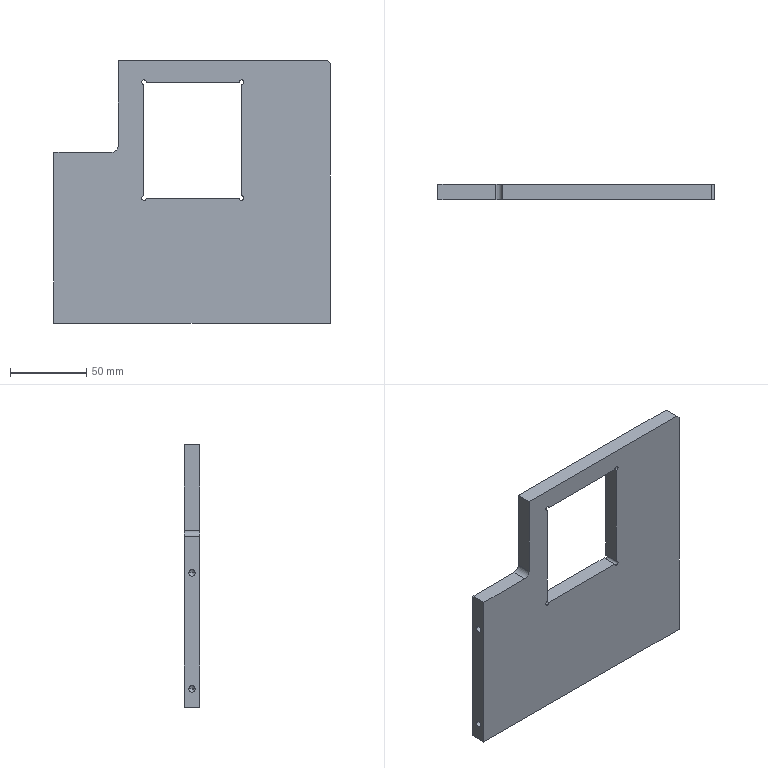Component | SolidWorks | AssemblyCylinderBracket54-1_GuideRailPlane-1 | 1 solid | 36 faces | box 181 x 10 x 172 mm | volume 236483 mm3 | cylinder 15 | plane 13 | cone 8 | commonest cylinder face diameters 4.2 x8 3 x6 8 x1
build123d program:
from build123d import *

# Parameters (mm, degrees)
SKETCH1_W                      = 172
SKETCH1_H                      = 181
BOSS_EXTRUDE1_DEPTH            = 10
CHAMFER1_SIZE                  = 2
M5X0_8_TAPPED_HOLE1_AT_2_COUNT = 2
M5X0_8_TAPPED_HOLE1_AT_2_PITCH = 76
SKETCH13_W                     = 60
SKETCH13_H                     = 42
CUT_EXTRUDE1_DEPTH             = 10
FILLET1_R                      = 4
SKETCH14_W                     = 76
SKETCH14_H                     = 64
CUT_EXTRUDE2_DEPTH             = 126.245
SKETCH15_R                     = 1.5
CUT_EXTRUDE3_DEPTH             = 10


with BuildPart() as part:
    # Sketch1 → Boss-Extrude1 (new body)
    with BuildSketch(Plane.XY):
        Rectangle(SKETCH1_W, SKETCH1_H)
    extrude(amount=BOSS_EXTRUDE1_DEPTH)

    # Chamfer1
    chamfer1_edges = [part.edges().sort_by_distance(p)[0] for p in [
        (86, -90.5, 5),
        (86, 90.5, 5),
    ]]
    chamfer(chamfer1_edges, length=CHAMFER1_SIZE)

    # Sketch6 → M5x0.8 Tapped Hole1 (revolve, cut)
    with BuildSketch(Plane(origin=(-74, -90.5, 5), x_dir=(0, 0, -1), z_dir=(1, 0, 0))):
        Polygon((0, 0), (0, 15.262), (2.1, 14), (2.1, 0), align=None)
    m5x0_8_tapped_hole1 = revolve(axis=Axis((-74, -96.85, 5), (0, 1, 0)), mode=Mode.SUBTRACT)

    # M5x0.8 Tapped Hole1 at 2: M5x0.8 Tapped Hole1 ×2
    with Locations(*[(i * M5X0_8_TAPPED_HOLE1_AT_2_PITCH, 0, 0) for i in range(1, M5X0_8_TAPPED_HOLE1_AT_2_COUNT)]):
        add(m5x0_8_tapped_hole1, mode=Mode.SUBTRACT)

    # Mirror1: M5x0.8 Tapped Hole1 across plane
    add(m5x0_8_tapped_hole1.mirror(Plane.ZX), mode=Mode.SUBTRACT)

    # Mirror1 copy 1 sketch → Mirror1 copy 1 (revolve, cut)
    with BuildSketch(Plane(origin=(2, 90.5, 5), x_dir=(0, 0, -1), z_dir=(1, 0, 0))):
        Polygon((0, 0), (0, -15.262), (2.1, -14), (2.1, 0), align=None)
    revolve(axis=Axis((2, 96.85, 5), (0, 1, 0)), mode=Mode.SUBTRACT)

    # Sketch13 → Cut-Extrude1 (cut)
    with BuildSketch(Plane.XY.offset(10)):
        with Locations((56, -69.5)):
            Rectangle(SKETCH13_W, SKETCH13_H)
    extrude(amount=-CUT_EXTRUDE1_DEPTH, mode=Mode.SUBTRACT)

    # Fillet1
    fillet1_edges = [part.edges().sort_by_distance(p)[0] for p in [
        (26, -48.5, 5),
    ]]
    fillet(fillet1_edges, radius=FILLET1_R)

    # Sketch14 → Cut-Extrude2 (cut, through all)
    with BuildSketch(Plane.XY.offset(10)):
        with Locations((34, 0.5)):
            Rectangle(SKETCH14_W, SKETCH14_H)
    extrude(amount=-CUT_EXTRUDE2_DEPTH, mode=Mode.SUBTRACT)

    # Sketch15 → Cut-Extrude3 (cut)
    with BuildSketch(Plane.XY.offset(10)):
        with Locations((-4, 32.5)):
            Circle(SKETCH15_R)
        with Locations((72, 32.5)):
            Circle(SKETCH15_R)
        with Locations((72, -31.5)):
            Circle(SKETCH15_R)
        with Locations((-4, -31.5)):
            Circle(SKETCH15_R)
    extrude(amount=-CUT_EXTRUDE3_DEPTH, mode=Mode.SUBTRACT)


solid = part.part

# Placed as in the assembly
solid = solid.moved(Location((54.585, -11.305, 87.359), (-90, 0, -90)))
STEP:
#1=COLOUR_RGB('',0.7922,0.8196,0.9333);
#2=FILL_AREA_STYLE_COLOUR('',#1);
#3=FILL_AREA_STYLE('',(#2));
#4=SURFACE_STYLE_FILL_AREA(#3);
#5=SURFACE_SIDE_STYLE('',(#4));
#6=SURFACE_STYLE_USAGE(.BOTH.,#5);
#7=PRESENTATION_STYLE_ASSIGNMENT((#6));
#8=CARTESIAN_POINT('',(0.9089,-0.4451,6.333));
#9=VERTEX_POINT('',#8);
#10=CARTESIAN_POINT('',(0.9679,-0.4451,6.274));
#11=VERTEX_POINT('',#10);
#12=CARTESIAN_POINT('',(0.9089,-0.4451,6.274));
#13=DIRECTION('',(-0.,1.,-0.));
#14=DIRECTION('',(0.,0.,1.));
#15=AXIS2_PLACEMENT_3D('',#12,#13,#14);
#16=CIRCLE('',#15,0.05906);
#17=EDGE_CURVE('',#9,#11,#16,.T.);
#18=ORIENTED_EDGE('',*,*,#17,.F.);
#19=CARTESIAN_POINT('',(0.9089,-0.05139,6.333));
#20=VERTEX_POINT('',#19);
#21=CARTESIAN_POINT('',(0.9089,-0.4451,6.333));
#22=DIRECTION('',(-0.,1.,-0.));
#23=VECTOR('',#22,39.37);
#24=LINE('',#21,#23);
#25=EDGE_CURVE('',#9,#20,#24,.T.);
#26=ORIENTED_EDGE('',*,*,#25,.T.);
#27=CARTESIAN_POINT('',(0.9679,-0.05139,6.274));
#28=VERTEX_POINT('',#27);
#29=CARTESIAN_POINT('',(0.9089,-0.05139,6.274));
#30=DIRECTION('',(-0.,1.,-0.));
#31=DIRECTION('',(0.,0.,1.));
#32=AXIS2_PLACEMENT_3D('',#29,#30,#31);
#33=CIRCLE('',#32,0.05906);
#34=EDGE_CURVE('',#20,#28,#33,.T.);
#35=ORIENTED_EDGE('',*,*,#34,.T.);
#36=CARTESIAN_POINT('',(0.9679,-0.4451,6.274));
#37=DIRECTION('',(-0.,1.,-0.));
#38=VECTOR('',#37,39.37);
#39=LINE('',#36,#38);
#40=EDGE_CURVE('',#11,#28,#39,.T.);
#41=ORIENTED_EDGE('',*,*,#40,.F.);
#42=EDGE_LOOP('',(#18,#26,#35,#41));
#43=FACE_OUTER_BOUND('',#42,.T.);
#44=CARTESIAN_POINT('',(0.9089,-0.4451,6.274));
#45=DIRECTION('',(-0.,1.,-0.));
#46=DIRECTION('',(0.,0.,1.));
#47=AXIS2_PLACEMENT_3D('',#44,#45,#46);
#48=CYLINDRICAL_SURFACE('',#47,0.05906);
#49=ADVANCED_FACE('',(#43),#48,.F.);
#50=CARTESIAN_POINT('',(3.429,-0.4451,6.333));
#51=VERTEX_POINT('',#50);
#52=CARTESIAN_POINT('',(3.429,-0.4451,6.215));
#53=VERTEX_POINT('',#52);
#54=CARTESIAN_POINT('',(3.429,-0.4451,6.274));
#55=DIRECTION('',(-0.,1.,-0.));
#56=DIRECTION('',(0.,0.,1.));
#57=AXIS2_PLACEMENT_3D('',#54,#55,#56);
#58=CIRCLE('',#57,0.05906);
#59=EDGE_CURVE('',#51,#53,#58,.T.);
#60=ORIENTED_EDGE('',*,*,#59,.F.);
#61=CARTESIAN_POINT('',(3.429,-0.05139,6.333));
#62=VERTEX_POINT('',#61);
#63=CARTESIAN_POINT('',(3.429,-0.4451,6.333));
#64=DIRECTION('',(-0.,1.,-0.));
#65=VECTOR('',#64,39.37);
#66=LINE('',#63,#65);
#67=EDGE_CURVE('',#51,#62,#66,.T.);
#68=ORIENTED_EDGE('',*,*,#67,.T.);
#69=CARTESIAN_POINT('',(3.429,-0.05139,6.215));
#70=VERTEX_POINT('',#69);
#71=CARTESIAN_POINT('',(3.429,-0.05139,6.274));
#72=DIRECTION('',(-0.,1.,-0.));
#73=DIRECTION('',(0.,0.,1.));
#74=AXIS2_PLACEMENT_3D('',#71,#72,#73);
#75=CIRCLE('',#74,0.05906);
#76=EDGE_CURVE('',#62,#70,#75,.T.);
#77=ORIENTED_EDGE('',*,*,#76,.T.);
#78=CARTESIAN_POINT('',(3.429,-0.4451,6.215));
#79=DIRECTION('',(-0.,1.,-0.));
#80=VECTOR('',#79,39.37);
#81=LINE('',#78,#80);
#82=EDGE_CURVE('',#53,#70,#81,.T.);
#83=ORIENTED_EDGE('',*,*,#82,.F.);
#84=EDGE_LOOP('',(#60,#68,#77,#83));
#85=FACE_OUTER_BOUND('',#84,.T.);
#86=CARTESIAN_POINT('',(3.429,-0.4451,6.274));
#87=DIRECTION('',(-0.,1.,-0.));
#88=DIRECTION('',(0.,0.,1.));
#89=AXIS2_PLACEMENT_3D('',#86,#87,#88);
#90=CYLINDRICAL_SURFACE('',#89,0.05906);
#91=ADVANCED_FACE('',(#85),#90,.F.);
#92=CARTESIAN_POINT('',(5.161,-0.3309,0.5259));
#93=VERTEX_POINT('',#92);
#94=CARTESIAN_POINT('',(5.161,-0.1656,0.5259));
#95=VERTEX_POINT('',#94);
#96=CARTESIAN_POINT('',(5.161,-0.2482,0.5259));
#97=DIRECTION('',(1.,-0.,0.));
#98=DIRECTION('',(0.,1.,0.));
#99=AXIS2_PLACEMENT_3D('',#96,#97,#98);
#100=CIRCLE('',#99,0.08268);
#101=EDGE_CURVE('',#93,#95,#100,.T.);
#102=ORIENTED_EDGE('',*,*,#101,.F.);
#103=CARTESIAN_POINT('',(5.712,-0.3309,0.5259));
#104=VERTEX_POINT('',#103);
#105=CARTESIAN_POINT('',(5.712,-0.3309,0.5259));
#106=DIRECTION('',(1.,-0.,0.));
#107=VECTOR('',#106,39.37);
#108=LINE('',#105,#107);
#109=EDGE_CURVE('',#93,#104,#108,.T.);
#110=ORIENTED_EDGE('',*,*,#109,.T.);
#111=CARTESIAN_POINT('',(5.712,-0.1656,0.5259));
#112=VERTEX_POINT('',#111);
#113=CARTESIAN_POINT('',(5.712,-0.2482,0.5259));
#114=DIRECTION('',(1.,-0.,0.));
#115=DIRECTION('',(0.,1.,0.));
#116=AXIS2_PLACEMENT_3D('',#113,#114,#115);
#117=CIRCLE('',#116,0.08268);
#118=EDGE_CURVE('',#104,#112,#117,.T.);
#119=ORIENTED_EDGE('',*,*,#118,.T.);
#120=CARTESIAN_POINT('',(5.712,-0.1656,0.5259));
#121=DIRECTION('',(1.,-0.,0.));
#122=VECTOR('',#121,39.37);
#123=LINE('',#120,#122);
#124=EDGE_CURVE('',#95,#112,#123,.T.);
#125=ORIENTED_EDGE('',*,*,#124,.F.);
#126=EDGE_LOOP('',(#102,#110,#119,#125));
#127=FACE_OUTER_BOUND('',#126,.T.);
#128=CARTESIAN_POINT('',(5.712,-0.2482,0.5259));
#129=DIRECTION('',(1.,-0.,0.));
#130=DIRECTION('',(0.,1.,0.));
#131=AXIS2_PLACEMENT_3D('',#128,#129,#130);
#132=CYLINDRICAL_SURFACE('',#131,0.08268);
#133=ADVANCED_FACE('',(#127),#132,.F.);
#134=CARTESIAN_POINT('',(5.111,-0.2482,0.5259));
#135=VERTEX_POINT('',#134);
#136=CARTESIAN_POINT('',(5.161,-0.1656,0.5259));
#137=DIRECTION('',(0.515,0.8572,0.));
#138=VECTOR('',#137,39.37);
#139=LINE('',#136,#138);
#140=EDGE_CURVE('',#135,#95,#139,.T.);
#141=ORIENTED_EDGE('',*,*,#140,.F.);
#142=CARTESIAN_POINT('',(5.161,-0.3309,0.5259));
#143=DIRECTION('',(0.515,-0.8572,0.));
#144=VECTOR('',#143,39.37);
#145=LINE('',#142,#144);
#146=EDGE_CURVE('',#135,#93,#145,.T.);
#147=ORIENTED_EDGE('',*,*,#146,.T.);
#148=ORIENTED_EDGE('',*,*,#101,.T.);
#149=EDGE_LOOP('',(#141,#147,#148));
#150=FACE_OUTER_BOUND('',#149,.T.);
#151=CARTESIAN_POINT('',(5.161,-0.2482,0.5259));
#152=DIRECTION('',(1.,-0.,0.));
#153=DIRECTION('',(0.,1.,0.));
#154=AXIS2_PLACEMENT_3D('',#151,#152,#153);
#155=CONICAL_SURFACE('',#154,0.08268,1.03);
#156=ADVANCED_FACE('',(#150),#155,.F.);
#157=CARTESIAN_POINT('',(5.161,-0.3309,3.518));
#158=VERTEX_POINT('',#157);
#159=CARTESIAN_POINT('',(5.161,-0.1656,3.518));
#160=VERTEX_POINT('',#159);
#161=CARTESIAN_POINT('',(5.161,-0.2482,3.518));
#162=DIRECTION('',(1.,-0.,0.));
#163=DIRECTION('',(0.,1.,0.));
#164=AXIS2_PLACEMENT_3D('',#161,#162,#163);
#165=CIRCLE('',#164,0.08268);
#166=EDGE_CURVE('',#158,#160,#165,.T.);
#167=ORIENTED_EDGE('',*,*,#166,.F.);
#168=CARTESIAN_POINT('',(5.712,-0.3309,3.518));
#169=VERTEX_POINT('',#168);
#170=CARTESIAN_POINT('',(5.712,-0.3309,3.518));
#171=DIRECTION('',(1.,-0.,0.));
#172=VECTOR('',#171,39.37);
#173=LINE('',#170,#172);
#174=EDGE_CURVE('',#158,#169,#173,.T.);
#175=ORIENTED_EDGE('',*,*,#174,.T.);
#176=CARTESIAN_POINT('',(5.712,-0.1656,3.518));
#177=VERTEX_POINT('',#176);
#178=CARTESIAN_POINT('',(5.712,-0.2482,3.518));
#179=DIRECTION('',(1.,-0.,0.));
#180=DIRECTION('',(0.,1.,0.));
#181=AXIS2_PLACEMENT_3D('',#178,#179,#180);
#182=CIRCLE('',#181,0.08268);
#183=EDGE_CURVE('',#169,#177,#182,.T.);
#184=ORIENTED_EDGE('',*,*,#183,.T.);
#185=CARTESIAN_POINT('',(5.712,-0.1656,3.518));
#186=DIRECTION('',(1.,-0.,0.));
#187=VECTOR('',#186,39.37);
#188=LINE('',#185,#187);
#189=EDGE_CURVE('',#160,#177,#188,.T.);
#190=ORIENTED_EDGE('',*,*,#189,.F.);
#191=EDGE_LOOP('',(#167,#175,#184,#190));
#192=FACE_OUTER_BOUND('',#191,.T.);
#193=CARTESIAN_POINT('',(5.712,-0.2482,3.518));
#194=DIRECTION('',(1.,-0.,0.));
#195=DIRECTION('',(0.,1.,0.));
#196=AXIS2_PLACEMENT_3D('',#193,#194,#195);
#197=CYLINDRICAL_SURFACE('',#196,0.08268);
#198=ADVANCED_FACE('',(#192),#197,.F.);
#199=CARTESIAN_POINT('',(5.111,-0.2482,3.518));
#200=VERTEX_POINT('',#199);
#201=CARTESIAN_POINT('',(5.161,-0.1656,3.518));
#202=DIRECTION('',(0.515,0.8572,0.));
#203=VECTOR('',#202,39.37);
#204=LINE('',#201,#203);
#205=EDGE_CURVE('',#200,#160,#204,.T.);
#206=ORIENTED_EDGE('',*,*,#205,.F.);
#207=CARTESIAN_POINT('',(5.161,-0.3309,3.518));
#208=DIRECTION('',(0.515,-0.8572,0.));
#209=VECTOR('',#208,39.37);
#210=LINE('',#207,#209);
#211=EDGE_CURVE('',#200,#158,#210,.T.);
#212=ORIENTED_EDGE('',*,*,#211,.T.);
#213=ORIENTED_EDGE('',*,*,#166,.T.);
#214=EDGE_LOOP('',(#206,#212,#213));
#215=FACE_OUTER_BOUND('',#214,.T.);
#216=CARTESIAN_POINT('',(5.161,-0.2482,3.518));
#217=DIRECTION('',(1.,-0.,0.));
#218=DIRECTION('',(0.,1.,0.));
#219=AXIS2_PLACEMENT_3D('',#216,#217,#218);
#220=CONICAL_SURFACE('',#219,0.08268,1.03);
#221=ADVANCED_FACE('',(#215),#220,.F.);
#222=CARTESIAN_POINT('',(-0.8628,-0.1656,0.5259));
#223=VERTEX_POINT('',#222);
#224=CARTESIAN_POINT('',(-0.8628,-0.3309,0.5259));
#225=VERTEX_POINT('',#224);
#226=CARTESIAN_POINT('',(-0.8628,-0.2482,0.5259));
#227=DIRECTION('',(-1.,0.,-0.));
#228=DIRECTION('',(0.,-1.,0.));
#229=AXIS2_PLACEMENT_3D('',#226,#227,#228);
#230=CIRCLE('',#229,0.08268);
#231=EDGE_CURVE('',#223,#225,#230,.T.);
#232=ORIENTED_EDGE('',*,*,#231,.F.);
#233=CARTESIAN_POINT('',(-1.414,-0.1656,0.5259));
#234=VERTEX_POINT('',#233);
#235=CARTESIAN_POINT('',(-1.414,-0.1656,0.5259));
#236=DIRECTION('',(-1.,0.,-0.));
#237=VECTOR('',#236,39.37);
#238=LINE('',#235,#237);
#239=EDGE_CURVE('',#223,#234,#238,.T.);
#240=ORIENTED_EDGE('',*,*,#239,.T.);
#241=CARTESIAN_POINT('',(-1.414,-0.3309,0.5259));
#242=VERTEX_POINT('',#241);
#243=CARTESIAN_POINT('',(-1.414,-0.2482,0.5259));
#244=DIRECTION('',(-1.,0.,-0.));
#245=DIRECTION('',(0.,-1.,0.));
#246=AXIS2_PLACEMENT_3D('',#243,#244,#245);
#247=CIRCLE('',#246,0.08268);
#248=EDGE_CURVE('',#234,#242,#247,.T.);
#249=ORIENTED_EDGE('',*,*,#248,.T.);
#250=CARTESIAN_POINT('',(-1.414,-0.3309,0.5259));
#251=DIRECTION('',(-1.,0.,-0.));
#252=VECTOR('',#251,39.37);
#253=LINE('',#250,#252);
#254=EDGE_CURVE('',#225,#242,#253,.T.);
#255=ORIENTED_EDGE('',*,*,#254,.F.);
#256=EDGE_LOOP('',(#232,#240,#249,#255));
#257=FACE_OUTER_BOUND('',#256,.T.);
#258=CARTESIAN_POINT('',(-1.414,-0.2482,0.5259));
#259=DIRECTION('',(-1.,0.,-0.));
#260=DIRECTION('',(0.,-1.,0.));
#261=AXIS2_PLACEMENT_3D('',#258,#259,#260);
#262=CYLINDRICAL_SURFACE('',#261,0.08268);
#263=ADVANCED_FACE('',(#257),#262,.F.);
#264=CARTESIAN_POINT('',(-0.8131,-0.2482,0.5259));
#265=VERTEX_POINT('',#264);
#266=CARTESIAN_POINT('',(-0.8628,-0.3309,0.5259));
#267=DIRECTION('',(-0.515,-0.8572,-0.));
#268=VECTOR('',#267,39.37);
#269=LINE('',#266,#268);
#270=EDGE_CURVE('',#265,#225,#269,.T.);
#271=ORIENTED_EDGE('',*,*,#270,.F.);
#272=CARTESIAN_POINT('',(-0.8628,-0.1656,0.5259));
#273=DIRECTION('',(-0.515,0.8572,0.));
#274=VECTOR('',#273,39.37);
#275=LINE('',#272,#274);
#276=EDGE_CURVE('',#265,#223,#275,.T.);
#277=ORIENTED_EDGE('',*,*,#276,.T.);
#278=ORIENTED_EDGE('',*,*,#231,.T.);
#279=EDGE_LOOP('',(#271,#277,#278));
#280=FACE_OUTER_BOUND('',#279,.T.);
#281=CARTESIAN_POINT('',(-0.8628,-0.2482,0.5259));
#282=DIRECTION('',(-1.,0.,-0.));
#283=DIRECTION('',(0.,-1.,0.));
#284=AXIS2_PLACEMENT_3D('',#281,#282,#283);
#285=CONICAL_SURFACE('',#284,0.08268,1.03);
#286=ADVANCED_FACE('',(#280),#285,.F.);
#287=CARTESIAN_POINT('',(-0.8628,-0.1656,3.518));
#288=VERTEX_POINT('',#287);
#289=CARTESIAN_POINT('',(-0.8628,-0.3309,3.518));
#290=VERTEX_POINT('',#289);
#291=CARTESIAN_POINT('',(-0.8628,-0.2482,3.518));
#292=DIRECTION('',(-1.,0.,-0.));
#293=DIRECTION('',(0.,-1.,0.));
#294=AXIS2_PLACEMENT_3D('',#291,#292,#293);
#295=CIRCLE('',#294,0.08268);
#296=EDGE_CURVE('',#288,#290,#295,.T.);
#297=ORIENTED_EDGE('',*,*,#296,.F.);
#298=CARTESIAN_POINT('',(-1.414,-0.1656,3.518));
#299=VERTEX_POINT('',#298);
#300=CARTESIAN_POINT('',(-1.414,-0.1656,3.518));
#301=DIRECTION('',(-1.,0.,-0.));
#302=VECTOR('',#301,39.37);
#303=LINE('',#300,#302);
#304=EDGE_CURVE('',#288,#299,#303,.T.);
#305=ORIENTED_EDGE('',*,*,#304,.T.);
#306=CARTESIAN_POINT('',(-1.414,-0.3309,3.518));
#307=VERTEX_POINT('',#306);
#308=CARTESIAN_POINT('',(-1.414,-0.2482,3.518));
#309=DIRECTION('',(-1.,0.,-0.));
#310=DIRECTION('',(0.,-1.,0.));
#311=AXIS2_PLACEMENT_3D('',#308,#309,#310);
#312=CIRCLE('',#311,0.08268);
#313=EDGE_CURVE('',#299,#307,#312,.T.);
#314=ORIENTED_EDGE('',*,*,#313,.T.);
#315=CARTESIAN_POINT('',(-1.414,-0.3309,3.518));
#316=DIRECTION('',(-1.,0.,-0.));
#317=VECTOR('',#316,39.37);
#318=LINE('',#315,#317);
#319=EDGE_CURVE('',#290,#307,#318,.T.);
#320=ORIENTED_EDGE('',*,*,#319,.F.);
#321=EDGE_LOOP('',(#297,#305,#314,#320));
#322=FACE_OUTER_BOUND('',#321,.T.);
#323=CARTESIAN_POINT('',(-1.414,-0.2482,3.518));
#324=DIRECTION('',(-1.,0.,-0.));
#325=DIRECTION('',(0.,-1.,0.));
#326=AXIS2_PLACEMENT_3D('',#323,#324,#325);
#327=CYLINDRICAL_SURFACE('',#326,0.08268);
#328=ADVANCED_FACE('',(#322),#327,.F.);
#329=CARTESIAN_POINT('',(-0.8131,-0.2482,3.518));
#330=VERTEX_POINT('',#329);
#331=CARTESIAN_POINT('',(-0.8628,-0.3309,3.518));
#332=DIRECTION('',(-0.515,-0.8572,-0.));
#333=VECTOR('',#332,39.37);
#334=LINE('',#331,#333);
#335=EDGE_CURVE('',#330,#290,#334,.T.);
#336=ORIENTED_EDGE('',*,*,#335,.F.);
#337=CARTESIAN_POINT('',(-0.8628,-0.1656,3.518));
#338=DIRECTION('',(-0.515,0.8572,0.));
#339=VECTOR('',#338,39.37);
#340=LINE('',#337,#339);
#341=EDGE_CURVE('',#330,#288,#340,.T.);
#342=ORIENTED_EDGE('',*,*,#341,.T.);
#343=ORIENTED_EDGE('',*,*,#296,.T.);
#344=EDGE_LOOP('',(#336,#342,#343));
#345=FACE_OUTER_BOUND('',#344,.T.);
#346=CARTESIAN_POINT('',(-0.8628,-0.2482,3.518));
#347=DIRECTION('',(-1.,0.,-0.));
#348=DIRECTION('',(0.,-1.,0.));
#349=AXIS2_PLACEMENT_3D('',#346,#347,#348);
#350=CONICAL_SURFACE('',#349,0.08268,1.03);
#351=ADVANCED_FACE('',(#345),#350,.F.);
#352=CARTESIAN_POINT('',(0.2396,-0.05139,6.825));
#353=VERTEX_POINT('',#352);
#354=CARTESIAN_POINT('',(5.633,-0.05139,6.825));
#355=VERTEX_POINT('',#354);
#356=CARTESIAN_POINT('',(5.712,-0.05139,6.825));
#357=DIRECTION('',(1.,-0.,-0.));
#358=VECTOR('',#357,39.37);
#359=LINE('',#356,#358);
#360=EDGE_CURVE('',#353,#355,#359,.T.);
#361=ORIENTED_EDGE('',*,*,#360,.F.);
#362=CARTESIAN_POINT('',(0.2396,-0.4451,6.825));
#363=VERTEX_POINT('',#362);
#364=CARTESIAN_POINT('',(0.2396,-0.4451,6.825));
#365=DIRECTION('',(-0.,1.,-0.));
#366=VECTOR('',#365,39.37);
#367=LINE('',#364,#366);
#368=EDGE_CURVE('',#363,#353,#367,.T.);
#369=ORIENTED_EDGE('',*,*,#368,.F.);
#370=CARTESIAN_POINT('',(5.633,-0.4451,6.825));
#371=VERTEX_POINT('',#370);
#372=CARTESIAN_POINT('',(5.712,-0.4451,6.825));
#373=DIRECTION('',(1.,-0.,-0.));
#374=VECTOR('',#373,39.37);
#375=LINE('',#372,#374);
#376=EDGE_CURVE('',#363,#371,#375,.T.);
#377=ORIENTED_EDGE('',*,*,#376,.T.);
#378=CARTESIAN_POINT('',(5.633,-0.05139,6.825));
#379=DIRECTION('',(-0.,1.,-0.));
#380=VECTOR('',#379,39.37);
#381=LINE('',#378,#380);
#382=EDGE_CURVE('',#371,#355,#381,.T.);
#383=ORIENTED_EDGE('',*,*,#382,.T.);
#384=EDGE_LOOP('',(#361,#369,#377,#383));
#385=FACE_OUTER_BOUND('',#384,.T.);
#386=CARTESIAN_POINT('',(5.712,-0.05139,6.825));
#387=DIRECTION('',(-0.,0.,-1.));
#388=DIRECTION('',(-1.,0.,0.));
#389=AXIS2_PLACEMENT_3D('',#386,#387,#388);
#390=PLANE('',#389);
#391=ADVANCED_FACE('',(#385),#390,.F.);
#392=CARTESIAN_POINT('',(5.712,-0.2482,0.5259));
#393=DIRECTION('',(1.,-0.,0.));
#394=DIRECTION('',(0.,1.,0.));
#395=AXIS2_PLACEMENT_3D('',#392,#393,#394);
#396=CIRCLE('',#395,0.08268);
#397=EDGE_CURVE('',#112,#104,#396,.T.);
#398=ORIENTED_EDGE('',*,*,#397,.F.);
#399=ORIENTED_EDGE('',*,*,#118,.F.);
#400=EDGE_LOOP('',(#398,#399));
#401=FACE_BOUND('',#400,.T.);
#402=CARTESIAN_POINT('',(5.712,-0.2482,3.518));
#403=DIRECTION('',(1.,-0.,0.));
#404=DIRECTION('',(0.,1.,0.));
#405=AXIS2_PLACEMENT_3D('',#402,#403,#404);
#406=CIRCLE('',#405,0.08268);
#407=EDGE_CURVE('',#177,#169,#406,.T.);
#408=ORIENTED_EDGE('',*,*,#407,.F.);
#409=ORIENTED_EDGE('',*,*,#183,.F.);
#410=EDGE_LOOP('',(#408,#409));
#411=FACE_BOUND('',#410,.T.);
#412=CARTESIAN_POINT('',(5.712,-0.05139,6.746));
#413=VERTEX_POINT('',#412);
#414=CARTESIAN_POINT('',(5.712,-0.05139,0.0535));
#415=VERTEX_POINT('',#414);
#416=CARTESIAN_POINT('',(5.712,-0.05139,0.0535));
#417=DIRECTION('',(0.,0.,-1.));
#418=VECTOR('',#417,39.37);
#419=LINE('',#416,#418);
#420=EDGE_CURVE('',#413,#415,#419,.T.);
#421=ORIENTED_EDGE('',*,*,#420,.F.);
#422=CARTESIAN_POINT('',(5.712,-0.4451,6.746));
#423=VERTEX_POINT('',#422);
#424=CARTESIAN_POINT('',(5.712,-0.05139,6.746));
#425=DIRECTION('',(0.,-1.,0.));
#426=VECTOR('',#425,39.37);
#427=LINE('',#424,#426);
#428=EDGE_CURVE('',#413,#423,#427,.T.);
#429=ORIENTED_EDGE('',*,*,#428,.T.);
#430=CARTESIAN_POINT('',(5.712,-0.4451,0.0535));
#431=VERTEX_POINT('',#430);
#432=CARTESIAN_POINT('',(5.712,-0.4451,0.0535));
#433=DIRECTION('',(0.,0.,-1.));
#434=VECTOR('',#433,39.37);
#435=LINE('',#432,#434);
#436=EDGE_CURVE('',#423,#431,#435,.T.);
#437=ORIENTED_EDGE('',*,*,#436,.T.);
#438=CARTESIAN_POINT('',(5.712,-0.05139,0.0535));
#439=DIRECTION('',(0.,-1.,0.));
#440=VECTOR('',#439,39.37);
#441=LINE('',#438,#440);
#442=EDGE_CURVE('',#415,#431,#441,.T.);
#443=ORIENTED_EDGE('',*,*,#442,.F.);
#444=EDGE_LOOP('',(#421,#429,#437,#443));
#445=FACE_OUTER_BOUND('',#444,.T.);
#446=CARTESIAN_POINT('',(5.712,-0.05139,0.0535));
#447=DIRECTION('',(-1.,-0.,-0.));
#448=DIRECTION('',(0.,-1.,0.));
#449=AXIS2_PLACEMENT_3D('',#446,#447,#448);
#450=PLANE('',#449);
#451=ADVANCED_FACE('',(#401,#411,#445),#450,.F.);
#452=CARTESIAN_POINT('',(-1.414,-0.4451,0.0535));
#453=VERTEX_POINT('',#452);
#454=CARTESIAN_POINT('',(5.712,-0.4451,0.0535));
#455=DIRECTION('',(-1.,0.,0.));
#456=VECTOR('',#455,39.37);
#457=LINE('',#454,#456);
#458=EDGE_CURVE('',#431,#453,#457,.T.);
#459=ORIENTED_EDGE('',*,*,#458,.T.);
#460=CARTESIAN_POINT('',(-1.414,-0.05139,0.0535));
#461=VERTEX_POINT('',#460);
#462=CARTESIAN_POINT('',(-1.414,-0.05139,0.0535));
#463=DIRECTION('',(0.,-1.,0.));
#464=VECTOR('',#463,39.37);
#465=LINE('',#462,#464);
#466=EDGE_CURVE('',#461,#453,#465,.T.);
#467=ORIENTED_EDGE('',*,*,#466,.F.);
#468=CARTESIAN_POINT('',(5.712,-0.05139,0.0535));
#469=DIRECTION('',(-1.,0.,0.));
#470=VECTOR('',#469,39.37);
#471=LINE('',#468,#470);
#472=EDGE_CURVE('',#415,#461,#471,.T.);
#473=ORIENTED_EDGE('',*,*,#472,.F.);
#474=ORIENTED_EDGE('',*,*,#442,.T.);
#475=EDGE_LOOP('',(#459,#467,#473,#474));
#476=FACE_OUTER_BOUND('',#475,.T.);
#477=CARTESIAN_POINT('',(5.712,-0.05139,0.0535));
#478=DIRECTION('',(0.,-0.,1.));
#479=DIRECTION('',(1.,-0.,-0.));
#480=AXIS2_PLACEMENT_3D('',#477,#478,#479);
#481=PLANE('',#480);
#482=ADVANCED_FACE('',(#476),#481,.F.);
#483=CARTESIAN_POINT('',(-1.414,-0.2482,0.5259));
#484=DIRECTION('',(-1.,0.,-0.));
#485=DIRECTION('',(0.,-1.,0.));
#486=AXIS2_PLACEMENT_3D('',#483,#484,#485);
#487=CIRCLE('',#486,0.08268);
#488=EDGE_CURVE('',#242,#234,#487,.T.);
#489=ORIENTED_EDGE('',*,*,#488,.F.);
#490=ORIENTED_EDGE('',*,*,#248,.F.);
#491=EDGE_LOOP('',(#489,#490));
#492=FACE_BOUND('',#491,.T.);
#493=CARTESIAN_POINT('',(-1.414,-0.2482,3.518));
#494=DIRECTION('',(-1.,0.,-0.));
#495=DIRECTION('',(0.,-1.,0.));
#496=AXIS2_PLACEMENT_3D('',#493,#494,#495);
#497=CIRCLE('',#496,0.08268);
#498=EDGE_CURVE('',#307,#299,#497,.T.);
#499=ORIENTED_EDGE('',*,*,#498,.F.);
#500=ORIENTED_EDGE('',*,*,#313,.F.);
#501=EDGE_LOOP('',(#499,#500));
#502=FACE_BOUND('',#501,.T.);
#503=CARTESIAN_POINT('',(-1.414,-0.4451,4.463));
#504=VERTEX_POINT('',#503);
#505=CARTESIAN_POINT('',(-1.414,-0.4451,0.0535));
#506=DIRECTION('',(-0.,-0.,1.));
#507=VECTOR('',#506,39.37);
#508=LINE('',#505,#507);
#509=EDGE_CURVE('',#453,#504,#508,.T.);
#510=ORIENTED_EDGE('',*,*,#509,.T.);
#511=CARTESIAN_POINT('',(-1.414,-0.05139,4.463));
#512=VERTEX_POINT('',#511);
#513=CARTESIAN_POINT('',(-1.414,-0.4451,4.463));
#514=DIRECTION('',(-0.,1.,-0.));
#515=VECTOR('',#514,39.37);
#516=LINE('',#513,#515);
#517=EDGE_CURVE('',#504,#512,#516,.T.);
#518=ORIENTED_EDGE('',*,*,#517,.T.);
#519=CARTESIAN_POINT('',(-1.414,-0.05139,0.0535));
#520=DIRECTION('',(-0.,-0.,1.));
#521=VECTOR('',#520,39.37);
#522=LINE('',#519,#521);
#523=EDGE_CURVE('',#461,#512,#522,.T.);
#524=ORIENTED_EDGE('',*,*,#523,.F.);
#525=ORIENTED_EDGE('',*,*,#466,.T.);
#526=EDGE_LOOP('',(#510,#518,#524,#525));
#527=FACE_OUTER_BOUND('',#526,.T.);
#528=CARTESIAN_POINT('',(-1.414,-0.05139,0.0535));
#529=DIRECTION('',(1.,0.,0.));
#530=DIRECTION('',(-0.,1.,-0.));
#531=AXIS2_PLACEMENT_3D('',#528,#529,#530);
#532=PLANE('',#531);
#533=ADVANCED_FACE('',(#492,#502,#527),#532,.F.);
#534=CARTESIAN_POINT('',(0.9679,-0.05139,3.282));
#535=VERTEX_POINT('',#534);
#536=CARTESIAN_POINT('',(0.9089,-0.05139,3.341));
#537=VERTEX_POINT('',#536);
#538=CARTESIAN_POINT('',(0.9089,-0.05139,3.282));
#539=DIRECTION('',(-0.,1.,-0.));
#540=DIRECTION('',(0.,0.,1.));
#541=AXIS2_PLACEMENT_3D('',#538,#539,#540);
#542=CIRCLE('',#541,0.05906);
#543=EDGE_CURVE('',#535,#537,#542,.T.);
#544=ORIENTED_EDGE('',*,*,#543,.F.);
#545=CARTESIAN_POINT('',(3.369,-0.05139,3.282));
#546=VERTEX_POINT('',#545);
#547=CARTESIAN_POINT('',(3.429,-0.05139,3.282));
#548=DIRECTION('',(-1.,0.,0.));
#549=VECTOR('',#548,39.37);
#550=LINE('',#547,#549);
#551=EDGE_CURVE('',#546,#535,#550,.T.);
#552=ORIENTED_EDGE('',*,*,#551,.F.);
#553=CARTESIAN_POINT('',(3.429,-0.05139,3.341));
#554=VERTEX_POINT('',#553);
#555=CARTESIAN_POINT('',(3.429,-0.05139,3.282));
#556=DIRECTION('',(-0.,1.,-0.));
#557=DIRECTION('',(0.,0.,1.));
#558=AXIS2_PLACEMENT_3D('',#555,#556,#557);
#559=CIRCLE('',#558,0.05906);
#560=EDGE_CURVE('',#554,#546,#559,.T.);
#561=ORIENTED_EDGE('',*,*,#560,.F.);
#562=CARTESIAN_POINT('',(3.429,-0.05139,6.274));
#563=DIRECTION('',(-0.,0.,-1.));
#564=VECTOR('',#563,39.37);
#565=LINE('',#562,#564);
#566=EDGE_CURVE('',#70,#554,#565,.T.);
#567=ORIENTED_EDGE('',*,*,#566,.F.);
#568=ORIENTED_EDGE('',*,*,#76,.F.);
#569=CARTESIAN_POINT('',(3.369,-0.05139,6.274));
#570=VERTEX_POINT('',#569);
#571=CARTESIAN_POINT('',(3.429,-0.05139,6.274));
#572=DIRECTION('',(-0.,1.,-0.));
#573=DIRECTION('',(0.,0.,1.));
#574=AXIS2_PLACEMENT_3D('',#571,#572,#573);
#575=CIRCLE('',#574,0.05906);
#576=EDGE_CURVE('',#570,#62,#575,.T.);
#577=ORIENTED_EDGE('',*,*,#576,.F.);
#578=CARTESIAN_POINT('',(3.429,-0.05139,6.274));
#579=DIRECTION('',(1.,-0.,-0.));
#580=VECTOR('',#579,39.37);
#581=LINE('',#578,#580);
#582=EDGE_CURVE('',#28,#570,#581,.T.);
#583=ORIENTED_EDGE('',*,*,#582,.F.);
#584=ORIENTED_EDGE('',*,*,#34,.F.);
#585=CARTESIAN_POINT('',(0.9089,-0.05139,6.215));
#586=VERTEX_POINT('',#585);
#587=CARTESIAN_POINT('',(0.9089,-0.05139,6.274));
#588=DIRECTION('',(-0.,1.,-0.));
#589=DIRECTION('',(0.,0.,1.));
#590=AXIS2_PLACEMENT_3D('',#587,#588,#589);
#591=CIRCLE('',#590,0.05906);
#592=EDGE_CURVE('',#586,#20,#591,.T.);
#593=ORIENTED_EDGE('',*,*,#592,.F.);
#594=CARTESIAN_POINT('',(0.9089,-0.05139,6.274));
#595=DIRECTION('',(0.,-0.,1.));
#596=VECTOR('',#595,39.37);
#597=LINE('',#594,#596);
#598=EDGE_CURVE('',#537,#586,#597,.T.);
#599=ORIENTED_EDGE('',*,*,#598,.F.);
#600=EDGE_LOOP('',(#544,#552,#561,#567,#568,#577,#583,#584,#593,#599));
#601=FACE_BOUND('',#600,.T.);
#602=CARTESIAN_POINT('',(0.08208,-0.05139,4.463));
#603=VERTEX_POINT('',#602);
#604=CARTESIAN_POINT('',(-1.414,-0.05139,4.463));
#605=DIRECTION('',(-1.,0.,-0.));
#606=VECTOR('',#605,39.37);
#607=LINE('',#604,#606);
#608=EDGE_CURVE('',#603,#512,#607,.T.);
#609=ORIENTED_EDGE('',*,*,#608,.F.);
#610=CARTESIAN_POINT('',(0.2396,-0.05139,4.62));
#611=VERTEX_POINT('',#610);
#612=CARTESIAN_POINT('',(0.08208,-0.05139,4.62));
#613=DIRECTION('',(0.,-1.,0.));
#614=DIRECTION('',(0.,0.,1.));
#615=AXIS2_PLACEMENT_3D('',#612,#613,#614);
#616=CIRCLE('',#615,0.1575);
#617=EDGE_CURVE('',#603,#611,#616,.T.);
#618=ORIENTED_EDGE('',*,*,#617,.T.);
#619=CARTESIAN_POINT('',(0.2396,-0.05139,6.825));
#620=DIRECTION('',(-0.,0.,-1.));
#621=VECTOR('',#620,39.37);
#622=LINE('',#619,#621);
#623=EDGE_CURVE('',#353,#611,#622,.T.);
#624=ORIENTED_EDGE('',*,*,#623,.F.);
#625=ORIENTED_EDGE('',*,*,#360,.T.);
#626=CARTESIAN_POINT('',(5.584,-0.05139,6.874));
#627=DIRECTION('',(0.7071,-0.,-0.7071));
#628=VECTOR('',#627,39.37);
#629=LINE('',#626,#628);
#630=EDGE_CURVE('',#355,#413,#629,.T.);
#631=ORIENTED_EDGE('',*,*,#630,.T.);
#632=ORIENTED_EDGE('',*,*,#420,.T.);
#633=ORIENTED_EDGE('',*,*,#472,.T.);
#634=ORIENTED_EDGE('',*,*,#523,.T.);
#635=EDGE_LOOP('',(#609,#618,#624,#625,#631,#632,#633,#634));
#636=FACE_OUTER_BOUND('',#635,.T.);
#637=CARTESIAN_POINT('',(2.149,-0.05139,3.439));
#638=DIRECTION('',(-0.,1.,0.));
#639=DIRECTION('',(-0.,-0.,1.));
#640=AXIS2_PLACEMENT_3D('',#637,#638,#639);
#641=PLANE('',#640);
#642=ADVANCED_FACE('',(#601,#636),#641,.T.);
#643=CARTESIAN_POINT('',(3.369,-0.4451,3.282));
#644=VERTEX_POINT('',#643);
#645=CARTESIAN_POINT('',(0.9679,-0.4451,3.282));
#646=VERTEX_POINT('',#645);
#647=CARTESIAN_POINT('',(3.429,-0.4451,3.282));
#648=DIRECTION('',(-1.,0.,0.));
#649=VECTOR('',#648,39.37);
#650=LINE('',#647,#649);
#651=EDGE_CURVE('',#644,#646,#650,.T.);
#652=ORIENTED_EDGE('',*,*,#651,.T.);
#653=CARTESIAN_POINT('',(0.9089,-0.4451,3.341));
#654=VERTEX_POINT('',#653);
#655=CARTESIAN_POINT('',(0.9089,-0.4451,3.282));
#656=DIRECTION('',(-0.,1.,-0.));
#657=DIRECTION('',(0.,0.,1.));
#658=AXIS2_PLACEMENT_3D('',#655,#656,#657);
#659=CIRCLE('',#658,0.05906);
#660=EDGE_CURVE('',#646,#654,#659,.T.);
#661=ORIENTED_EDGE('',*,*,#660,.T.);
#662=CARTESIAN_POINT('',(0.9089,-0.4451,6.215));
#663=VERTEX_POINT('',#662);
#664=CARTESIAN_POINT('',(0.9089,-0.4451,6.274));
#665=DIRECTION('',(0.,-0.,1.));
#666=VECTOR('',#665,39.37);
#667=LINE('',#664,#666);
#668=EDGE_CURVE('',#654,#663,#667,.T.);
#669=ORIENTED_EDGE('',*,*,#668,.T.);
#670=CARTESIAN_POINT('',(0.9089,-0.4451,6.274));
#671=DIRECTION('',(-0.,1.,-0.));
#672=DIRECTION('',(0.,0.,1.));
#673=AXIS2_PLACEMENT_3D('',#670,#671,#672);
#674=CIRCLE('',#673,0.05906);
#675=EDGE_CURVE('',#663,#9,#674,.T.);
#676=ORIENTED_EDGE('',*,*,#675,.T.);
#677=ORIENTED_EDGE('',*,*,#17,.T.);
#678=CARTESIAN_POINT('',(3.369,-0.4451,6.274));
#679=VERTEX_POINT('',#678);
#680=CARTESIAN_POINT('',(3.429,-0.4451,6.274));
#681=DIRECTION('',(1.,-0.,-0.));
#682=VECTOR('',#681,39.37);
#683=LINE('',#680,#682);
#684=EDGE_CURVE('',#11,#679,#683,.T.);
#685=ORIENTED_EDGE('',*,*,#684,.T.);
#686=CARTESIAN_POINT('',(3.429,-0.4451,6.274));
#687=DIRECTION('',(-0.,1.,-0.));
#688=DIRECTION('',(0.,0.,1.));
#689=AXIS2_PLACEMENT_3D('',#686,#687,#688);
#690=CIRCLE('',#689,0.05906);
#691=EDGE_CURVE('',#679,#51,#690,.T.);
#692=ORIENTED_EDGE('',*,*,#691,.T.);
#693=ORIENTED_EDGE('',*,*,#59,.T.);
#694=CARTESIAN_POINT('',(3.429,-0.4451,3.341));
#695=VERTEX_POINT('',#694);
#696=CARTESIAN_POINT('',(3.429,-0.4451,6.274));
#697=DIRECTION('',(-0.,0.,-1.));
#698=VECTOR('',#697,39.37);
#699=LINE('',#696,#698);
#700=EDGE_CURVE('',#53,#695,#699,.T.);
#701=ORIENTED_EDGE('',*,*,#700,.T.);
#702=CARTESIAN_POINT('',(3.429,-0.4451,3.282));
#703=DIRECTION('',(-0.,1.,-0.));
#704=DIRECTION('',(0.,0.,1.));
#705=AXIS2_PLACEMENT_3D('',#702,#703,#704);
#706=CIRCLE('',#705,0.05906);
#707=EDGE_CURVE('',#695,#644,#706,.T.);
#708=ORIENTED_EDGE('',*,*,#707,.T.);
#709=EDGE_LOOP('',(#652,#661,#669,#676,#677,#685,#692,#693,#701,#708));
#710=FACE_BOUND('',#709,.T.);
#711=CARTESIAN_POINT('',(0.2396,-0.4451,4.62));
#712=VERTEX_POINT('',#711);
#713=CARTESIAN_POINT('',(0.2396,-0.4451,6.825));
#714=DIRECTION('',(-0.,0.,-1.));
#715=VECTOR('',#714,39.37);
#716=LINE('',#713,#715);
#717=EDGE_CURVE('',#363,#712,#716,.T.);
#718=ORIENTED_EDGE('',*,*,#717,.T.);
#719=CARTESIAN_POINT('',(0.08208,-0.4451,4.463));
#720=VERTEX_POINT('',#719);
#721=CARTESIAN_POINT('',(0.08208,-0.4451,4.62));
#722=DIRECTION('',(-0.,1.,-0.));
#723=DIRECTION('',(-0.,0.,1.));
#724=AXIS2_PLACEMENT_3D('',#721,#722,#723);
#725=CIRCLE('',#724,0.1575);
#726=EDGE_CURVE('',#712,#720,#725,.T.);
#727=ORIENTED_EDGE('',*,*,#726,.T.);
#728=CARTESIAN_POINT('',(-1.414,-0.4451,4.463));
#729=DIRECTION('',(-1.,0.,-0.));
#730=VECTOR('',#729,39.37);
#731=LINE('',#728,#730);
#732=EDGE_CURVE('',#720,#504,#731,.T.);
#733=ORIENTED_EDGE('',*,*,#732,.T.);
#734=ORIENTED_EDGE('',*,*,#509,.F.);
#735=ORIENTED_EDGE('',*,*,#458,.F.);
#736=ORIENTED_EDGE('',*,*,#436,.F.);
#737=CARTESIAN_POINT('',(5.712,-0.4451,6.746));
#738=DIRECTION('',(-0.7071,0.,0.7071));
#739=VECTOR('',#738,39.37);
#740=LINE('',#737,#739);
#741=EDGE_CURVE('',#423,#371,#740,.T.);
#742=ORIENTED_EDGE('',*,*,#741,.T.);
#743=ORIENTED_EDGE('',*,*,#376,.F.);
#744=EDGE_LOOP('',(#718,#727,#733,#734,#735,#736,#742,#743));
#745=FACE_OUTER_BOUND('',#744,.T.);
#746=CARTESIAN_POINT('',(2.149,-0.4451,3.439));
#747=DIRECTION('',(-0.,1.,0.));
#748=DIRECTION('',(-0.,-0.,1.));
#749=AXIS2_PLACEMENT_3D('',#746,#747,#748);
#750=PLANE('',#749);
#751=ADVANCED_FACE('',(#710,#745),#750,.F.);
#752=ORIENTED_EDGE('',*,*,#630,.F.);
#753=ORIENTED_EDGE('',*,*,#382,.F.);
#754=ORIENTED_EDGE('',*,*,#741,.F.);
#755=ORIENTED_EDGE('',*,*,#428,.F.);
#756=EDGE_LOOP('',(#752,#753,#754,#755));
#757=FACE_OUTER_BOUND('',#756,.T.);
#758=CARTESIAN_POINT('',(5.712,-0.05139,6.746));
#759=DIRECTION('',(-0.7071,-0.,-0.7071));
#760=DIRECTION('',(0.,-1.,0.));
#761=AXIS2_PLACEMENT_3D('',#758,#759,#760);
#762=PLANE('',#761);
#763=ADVANCED_FACE('',(#757),#762,.F.);
#764=ORIENTED_EDGE('',*,*,#341,.F.);
#765=ORIENTED_EDGE('',*,*,#335,.T.);
#766=CARTESIAN_POINT('',(-0.8628,-0.2482,3.518));
#767=DIRECTION('',(-1.,0.,-0.));
#768=DIRECTION('',(0.,-1.,0.));
#769=AXIS2_PLACEMENT_3D('',#766,#767,#768);
#770=CIRCLE('',#769,0.08268);
#771=EDGE_CURVE('',#290,#288,#770,.T.);
#772=ORIENTED_EDGE('',*,*,#771,.T.);
#773=EDGE_LOOP('',(#764,#765,#772));
#774=FACE_OUTER_BOUND('',#773,.T.);
#775=CARTESIAN_POINT('',(-0.8628,-0.2482,3.518));
#776=DIRECTION('',(-1.,0.,-0.));
#777=DIRECTION('',(0.,-1.,0.));
#778=AXIS2_PLACEMENT_3D('',#775,#776,#777);
#779=CONICAL_SURFACE('',#778,0.08268,1.03);
#780=ADVANCED_FACE('',(#774),#779,.F.);
#781=ORIENTED_EDGE('',*,*,#304,.F.);
#782=ORIENTED_EDGE('',*,*,#771,.F.);
#783=ORIENTED_EDGE('',*,*,#319,.T.);
#784=ORIENTED_EDGE('',*,*,#498,.T.);
#785=EDGE_LOOP('',(#781,#782,#783,#784));
#786=FACE_OUTER_BOUND('',#785,.T.);
#787=CARTESIAN_POINT('',(-1.414,-0.2482,3.518));
#788=DIRECTION('',(-1.,0.,-0.));
#789=DIRECTION('',(0.,-1.,0.));
#790=AXIS2_PLACEMENT_3D('',#787,#788,#789);
#791=CYLINDRICAL_SURFACE('',#790,0.08268);
#792=ADVANCED_FACE('',(#786),#791,.F.);
#793=ORIENTED_EDGE('',*,*,#276,.F.);
#794=ORIENTED_EDGE('',*,*,#270,.T.);
#795=CARTESIAN_POINT('',(-0.8628,-0.2482,0.5259));
#796=DIRECTION('',(-1.,0.,-0.));
#797=DIRECTION('',(0.,-1.,0.));
#798=AXIS2_PLACEMENT_3D('',#795,#796,#797);
#799=CIRCLE('',#798,0.08268);
#800=EDGE_CURVE('',#225,#223,#799,.T.);
#801=ORIENTED_EDGE('',*,*,#800,.T.);
#802=EDGE_LOOP('',(#793,#794,#801));
#803=FACE_OUTER_BOUND('',#802,.T.);
#804=CARTESIAN_POINT('',(-0.8628,-0.2482,0.5259));
#805=DIRECTION('',(-1.,0.,-0.));
#806=DIRECTION('',(0.,-1.,0.));
#807=AXIS2_PLACEMENT_3D('',#804,#805,#806);
#808=CONICAL_SURFACE('',#807,0.08268,1.03);
#809=ADVANCED_FACE('',(#803),#808,.F.);
#810=ORIENTED_EDGE('',*,*,#239,.F.);
#811=ORIENTED_EDGE('',*,*,#800,.F.);
#812=ORIENTED_EDGE('',*,*,#254,.T.);
#813=ORIENTED_EDGE('',*,*,#488,.T.);
#814=EDGE_LOOP('',(#810,#811,#812,#813));
#815=FACE_OUTER_BOUND('',#814,.T.);
#816=CARTESIAN_POINT('',(-1.414,-0.2482,0.5259));
#817=DIRECTION('',(-1.,0.,-0.));
#818=DIRECTION('',(0.,-1.,0.));
#819=AXIS2_PLACEMENT_3D('',#816,#817,#818);
#820=CYLINDRICAL_SURFACE('',#819,0.08268);
#821=ADVANCED_FACE('',(#815),#820,.F.);
#822=ORIENTED_EDGE('',*,*,#211,.F.);
#823=ORIENTED_EDGE('',*,*,#205,.T.);
#824=CARTESIAN_POINT('',(5.161,-0.2482,3.518));
#825=DIRECTION('',(1.,-0.,0.));
#826=DIRECTION('',(0.,1.,0.));
#827=AXIS2_PLACEMENT_3D('',#824,#825,#826);
#828=CIRCLE('',#827,0.08268);
#829=EDGE_CURVE('',#160,#158,#828,.T.);
#830=ORIENTED_EDGE('',*,*,#829,.T.);
#831=EDGE_LOOP('',(#822,#823,#830));
#832=FACE_OUTER_BOUND('',#831,.T.);
#833=CARTESIAN_POINT('',(5.161,-0.2482,3.518));
#834=DIRECTION('',(1.,-0.,0.));
#835=DIRECTION('',(0.,1.,0.));
#836=AXIS2_PLACEMENT_3D('',#833,#834,#835);
#837=CONICAL_SURFACE('',#836,0.08268,1.03);
#838=ADVANCED_FACE('',(#832),#837,.F.);
#839=ORIENTED_EDGE('',*,*,#174,.F.);
#840=ORIENTED_EDGE('',*,*,#829,.F.);
#841=ORIENTED_EDGE('',*,*,#189,.T.);
#842=ORIENTED_EDGE('',*,*,#407,.T.);
#843=EDGE_LOOP('',(#839,#840,#841,#842));
#844=FACE_OUTER_BOUND('',#843,.T.);
#845=CARTESIAN_POINT('',(5.712,-0.2482,3.518));
#846=DIRECTION('',(1.,-0.,0.));
#847=DIRECTION('',(0.,1.,0.));
#848=AXIS2_PLACEMENT_3D('',#845,#846,#847);
#849=CYLINDRICAL_SURFACE('',#848,0.08268);
#850=ADVANCED_FACE('',(#844),#849,.F.);
#851=ORIENTED_EDGE('',*,*,#146,.F.);
#852=ORIENTED_EDGE('',*,*,#140,.T.);
#853=CARTESIAN_POINT('',(5.161,-0.2482,0.5259));
#854=DIRECTION('',(1.,-0.,0.));
#855=DIRECTION('',(0.,1.,0.));
#856=AXIS2_PLACEMENT_3D('',#853,#854,#855);
#857=CIRCLE('',#856,0.08268);
#858=EDGE_CURVE('',#95,#93,#857,.T.);
#859=ORIENTED_EDGE('',*,*,#858,.T.);
#860=EDGE_LOOP('',(#851,#852,#859));
#861=FACE_OUTER_BOUND('',#860,.T.);
#862=CARTESIAN_POINT('',(5.161,-0.2482,0.5259));
#863=DIRECTION('',(1.,-0.,0.));
#864=DIRECTION('',(0.,1.,0.));
#865=AXIS2_PLACEMENT_3D('',#862,#863,#864);
#866=CONICAL_SURFACE('',#865,0.08268,1.03);
#867=ADVANCED_FACE('',(#861),#866,.F.);
#868=ORIENTED_EDGE('',*,*,#109,.F.);
#869=ORIENTED_EDGE('',*,*,#858,.F.);
#870=ORIENTED_EDGE('',*,*,#124,.T.);
#871=ORIENTED_EDGE('',*,*,#397,.T.);
#872=EDGE_LOOP('',(#868,#869,#870,#871));
#873=FACE_OUTER_BOUND('',#872,.T.);
#874=CARTESIAN_POINT('',(5.712,-0.2482,0.5259));
#875=DIRECTION('',(1.,-0.,0.));
#876=DIRECTION('',(0.,1.,0.));
#877=AXIS2_PLACEMENT_3D('',#874,#875,#876);
#878=CYLINDRICAL_SURFACE('',#877,0.08268);
#879=ADVANCED_FACE('',(#873),#878,.F.);
#880=ORIENTED_EDGE('',*,*,#732,.F.);
#881=CARTESIAN_POINT('',(0.08208,-0.05139,4.463));
#882=DIRECTION('',(-0.,1.,-0.));
#883=VECTOR('',#882,39.37);
#884=LINE('',#881,#883);
#885=EDGE_CURVE('',#720,#603,#884,.T.);
#886=ORIENTED_EDGE('',*,*,#885,.T.);
#887=ORIENTED_EDGE('',*,*,#608,.T.);
#888=ORIENTED_EDGE('',*,*,#517,.F.);
#889=EDGE_LOOP('',(#880,#886,#887,#888));
#890=FACE_OUTER_BOUND('',#889,.T.);
#891=CARTESIAN_POINT('',(-1.414,-0.4451,4.463));
#892=DIRECTION('',(0.,-0.,-1.));
#893=DIRECTION('',(-0.,1.,-0.));
#894=AXIS2_PLACEMENT_3D('',#891,#892,#893);
#895=PLANE('',#894);
#896=ADVANCED_FACE('',(#890),#895,.F.);
#897=ORIENTED_EDGE('',*,*,#623,.T.);
#898=CARTESIAN_POINT('',(0.2396,-0.4451,4.62));
#899=DIRECTION('',(0.,-1.,0.));
#900=VECTOR('',#899,39.37);
#901=LINE('',#898,#900);
#902=EDGE_CURVE('',#611,#712,#901,.T.);
#903=ORIENTED_EDGE('',*,*,#902,.T.);
#904=ORIENTED_EDGE('',*,*,#717,.F.);
#905=ORIENTED_EDGE('',*,*,#368,.T.);
#906=EDGE_LOOP('',(#897,#903,#904,#905));
#907=FACE_OUTER_BOUND('',#906,.T.);
#908=CARTESIAN_POINT('',(0.2396,-0.4451,6.825));
#909=DIRECTION('',(1.,-0.,-0.));
#910=DIRECTION('',(-0.,0.,-1.));
#911=AXIS2_PLACEMENT_3D('',#908,#909,#910);
#912=PLANE('',#911);
#913=ADVANCED_FACE('',(#907),#912,.F.);
#914=ORIENTED_EDGE('',*,*,#726,.F.);
#915=ORIENTED_EDGE('',*,*,#902,.F.);
#916=ORIENTED_EDGE('',*,*,#617,.F.);
#917=ORIENTED_EDGE('',*,*,#885,.F.);
#918=EDGE_LOOP('',(#914,#915,#916,#917));
#919=FACE_OUTER_BOUND('',#918,.T.);
#920=CARTESIAN_POINT('',(0.08208,-0.4451,4.62));
#921=DIRECTION('',(0.,-1.,0.));
#922=DIRECTION('',(0.,0.,-1.));
#923=AXIS2_PLACEMENT_3D('',#920,#921,#922);
#924=CYLINDRICAL_SURFACE('',#923,0.1575);
#925=ADVANCED_FACE('',(#919),#924,.F.);
#926=ORIENTED_EDGE('',*,*,#684,.F.);
#927=ORIENTED_EDGE('',*,*,#40,.T.);
#928=ORIENTED_EDGE('',*,*,#582,.T.);
#929=CARTESIAN_POINT('',(3.369,-0.4451,6.274));
#930=DIRECTION('',(0.,-1.,0.));
#931=VECTOR('',#930,39.37);
#932=LINE('',#929,#931);
#933=EDGE_CURVE('',#570,#679,#932,.T.);
#934=ORIENTED_EDGE('',*,*,#933,.T.);
#935=EDGE_LOOP('',(#926,#927,#928,#934));
#936=FACE_OUTER_BOUND('',#935,.T.);
#937=CARTESIAN_POINT('',(3.429,-0.4451,6.274));
#938=DIRECTION('',(0.,-0.,1.));
#939=DIRECTION('',(1.,-0.,-0.));
#940=AXIS2_PLACEMENT_3D('',#937,#938,#939);
#941=PLANE('',#940);
#942=ADVANCED_FACE('',(#936),#941,.F.);
#943=ORIENTED_EDGE('',*,*,#668,.F.);
#944=CARTESIAN_POINT('',(0.9089,-0.4451,3.341));
#945=DIRECTION('',(-0.,1.,-0.));
#946=VECTOR('',#945,39.37);
#947=LINE('',#944,#946);
#948=EDGE_CURVE('',#654,#537,#947,.T.);
#949=ORIENTED_EDGE('',*,*,#948,.T.);
#950=ORIENTED_EDGE('',*,*,#598,.T.);
#951=CARTESIAN_POINT('',(0.9089,-0.4451,6.215));
#952=DIRECTION('',(0.,-1.,0.));
#953=VECTOR('',#952,39.37);
#954=LINE('',#951,#953);
#955=EDGE_CURVE('',#586,#663,#954,.T.);
#956=ORIENTED_EDGE('',*,*,#955,.T.);
#957=EDGE_LOOP('',(#943,#949,#950,#956));
#958=FACE_OUTER_BOUND('',#957,.T.);
#959=CARTESIAN_POINT('',(0.9089,-0.4451,6.274));
#960=DIRECTION('',(-1.,0.,0.));
#961=DIRECTION('',(0.,-0.,1.));
#962=AXIS2_PLACEMENT_3D('',#959,#960,#961);
#963=PLANE('',#962);
#964=ADVANCED_FACE('',(#958),#963,.F.);
#965=ORIENTED_EDGE('',*,*,#551,.T.);
#966=CARTESIAN_POINT('',(0.9679,-0.4451,3.282));
#967=DIRECTION('',(0.,-1.,0.));
#968=VECTOR('',#967,39.37);
#969=LINE('',#966,#968);
#970=EDGE_CURVE('',#535,#646,#969,.T.);
#971=ORIENTED_EDGE('',*,*,#970,.T.);
#972=ORIENTED_EDGE('',*,*,#651,.F.);
#973=CARTESIAN_POINT('',(3.369,-0.4451,3.282));
#974=DIRECTION('',(-0.,1.,-0.));
#975=VECTOR('',#974,39.37);
#976=LINE('',#973,#975);
#977=EDGE_CURVE('',#644,#546,#976,.T.);
#978=ORIENTED_EDGE('',*,*,#977,.T.);
#979=EDGE_LOOP('',(#965,#971,#972,#978));
#980=FACE_OUTER_BOUND('',#979,.T.);
#981=CARTESIAN_POINT('',(3.429,-0.4451,3.282));
#982=DIRECTION('',(-0.,0.,-1.));
#983=DIRECTION('',(-1.,0.,0.));
#984=AXIS2_PLACEMENT_3D('',#981,#982,#983);
#985=PLANE('',#984);
#986=ADVANCED_FACE('',(#980),#985,.F.);
#987=ORIENTED_EDGE('',*,*,#700,.F.);
#988=ORIENTED_EDGE('',*,*,#82,.T.);
#989=ORIENTED_EDGE('',*,*,#566,.T.);
#990=CARTESIAN_POINT('',(3.429,-0.4451,3.341));
#991=DIRECTION('',(0.,-1.,0.));
#992=VECTOR('',#991,39.37);
#993=LINE('',#990,#992);
#994=EDGE_CURVE('',#554,#695,#993,.T.);
#995=ORIENTED_EDGE('',*,*,#994,.T.);
#996=EDGE_LOOP('',(#987,#988,#989,#995));
#997=FACE_OUTER_BOUND('',#996,.T.);
#998=CARTESIAN_POINT('',(3.429,-0.4451,6.274));
#999=DIRECTION('',(1.,-0.,-0.));
#1000=DIRECTION('',(-0.,0.,-1.));
#1001=AXIS2_PLACEMENT_3D('',#998,#999,#1000);
#1002=PLANE('',#1001);
#1003=ADVANCED_FACE('',(#997),#1002,.F.);
#1004=ORIENTED_EDGE('',*,*,#707,.F.);
#1005=ORIENTED_EDGE('',*,*,#994,.F.);
#1006=ORIENTED_EDGE('',*,*,#560,.T.);
#1007=ORIENTED_EDGE('',*,*,#977,.F.);
#1008=EDGE_LOOP('',(#1004,#1005,#1006,#1007));
#1009=FACE_OUTER_BOUND('',#1008,.T.);
#1010=CARTESIAN_POINT('',(3.429,-0.4451,3.282));
#1011=DIRECTION('',(-0.,1.,-0.));
#1012=DIRECTION('',(0.,0.,1.));
#1013=AXIS2_PLACEMENT_3D('',#1010,#1011,#1012);
#1014=CYLINDRICAL_SURFACE('',#1013,0.05906);
#1015=ADVANCED_FACE('',(#1009),#1014,.F.);
#1016=ORIENTED_EDGE('',*,*,#67,.F.);
#1017=ORIENTED_EDGE('',*,*,#691,.F.);
#1018=ORIENTED_EDGE('',*,*,#933,.F.);
#1019=ORIENTED_EDGE('',*,*,#576,.T.);
#1020=EDGE_LOOP('',(#1016,#1017,#1018,#1019));
#1021=FACE_OUTER_BOUND('',#1020,.T.);
#1022=CARTESIAN_POINT('',(3.429,-0.4451,6.274));
#1023=DIRECTION('',(-0.,1.,-0.));
#1024=DIRECTION('',(0.,0.,1.));
#1025=AXIS2_PLACEMENT_3D('',#1022,#1023,#1024);
#1026=CYLINDRICAL_SURFACE('',#1025,0.05906);
#1027=ADVANCED_FACE('',(#1021),#1026,.F.);
#1028=ORIENTED_EDGE('',*,*,#25,.F.);
#1029=ORIENTED_EDGE('',*,*,#675,.F.);
#1030=ORIENTED_EDGE('',*,*,#955,.F.);
#1031=ORIENTED_EDGE('',*,*,#592,.T.);
#1032=EDGE_LOOP('',(#1028,#1029,#1030,#1031));
#1033=FACE_OUTER_BOUND('',#1032,.T.);
#1034=CARTESIAN_POINT('',(0.9089,-0.4451,6.274));
#1035=DIRECTION('',(-0.,1.,-0.));
#1036=DIRECTION('',(0.,0.,1.));
#1037=AXIS2_PLACEMENT_3D('',#1034,#1035,#1036);
#1038=CYLINDRICAL_SURFACE('',#1037,0.05906);
#1039=ADVANCED_FACE('',(#1033),#1038,.F.);
#1040=ORIENTED_EDGE('',*,*,#660,.F.);
#1041=ORIENTED_EDGE('',*,*,#970,.F.);
#1042=ORIENTED_EDGE('',*,*,#543,.T.);
#1043=ORIENTED_EDGE('',*,*,#948,.F.);
#1044=EDGE_LOOP('',(#1040,#1041,#1042,#1043));
#1045=FACE_OUTER_BOUND('',#1044,.T.);
#1046=CARTESIAN_POINT('',(0.9089,-0.4451,3.282));
#1047=DIRECTION('',(-0.,1.,-0.));
#1048=DIRECTION('',(0.,0.,1.));
#1049=AXIS2_PLACEMENT_3D('',#1046,#1047,#1048);
#1050=CYLINDRICAL_SURFACE('',#1049,0.05906);
#1051=ADVANCED_FACE('',(#1045),#1050,.F.);
#1052=CLOSED_SHELL('',(#49,#91,#133,#156,#198,#221,#263,#286,#328,#351,#391,#451,#482,#533,#642,#751,#763,#780,#792,#809,#821,#838,#850,#867,#879,#896,#913,#925,#942,#964,#986,#1003,#1015,#1027,#1039,#1051));
#1053=MANIFOLD_SOLID_BREP('',#1052);
#1054=STYLED_ITEM('',(#7),#1053);
#1055=PRESENTATION_LAYER_ASSIGNMENT('','',(#1054));
#1056=(LENGTH_UNIT()NAMED_UNIT(*)SI_UNIT($,.METRE.));
#1057=LENGTH_MEASURE_WITH_UNIT(LENGTH_MEASURE(0.0254),#1056);
#1058=DIMENSIONAL_EXPONENTS(1.,0.,0.,0.,0.,0.,0.);
#1059=(CONVERSION_BASED_UNIT('',#1057)LENGTH_UNIT()NAMED_UNIT(#1058));
#1060=UNCERTAINTY_MEASURE_WITH_UNIT(LENGTH_MEASURE(0.00001),#1059,'','');
#1061=(NAMED_UNIT(*)PLANE_ANGLE_UNIT()SI_UNIT($,.RADIAN.));
#1062=(NAMED_UNIT(*)SI_UNIT($,.STERADIAN.)SOLID_ANGLE_UNIT());
#1063=(GEOMETRIC_REPRESENTATION_CONTEXT(3)GLOBAL_UNCERTAINTY_ASSIGNED_CONTEXT((#1060))GLOBAL_UNIT_ASSIGNED_CONTEXT((#1059,#1061,#1062))REPRESENTATION_CONTEXT('',''));
#1064=MECHANICAL_DESIGN_GEOMETRIC_PRESENTATION_REPRESENTATION('',(#1054),#1063);
#1065=CARTESIAN_POINT('',(0.,0.,0.));
#1066=DIRECTION('',(0.,0.,1.));
#1067=DIRECTION('',(1.,0.,0.));
#1068=AXIS2_PLACEMENT_3D('',#1065,#1066,#1067);
#1069=(LENGTH_UNIT()NAMED_UNIT(*)SI_UNIT($,.METRE.));
#1070=LENGTH_MEASURE_WITH_UNIT(LENGTH_MEASURE(0.0254),#1069);
#1071=DIMENSIONAL_EXPONENTS(1.,0.,0.,0.,0.,0.,0.);
#1072=(CONVERSION_BASED_UNIT('',#1070)LENGTH_UNIT()NAMED_UNIT(#1071));
#1073=UNCERTAINTY_MEASURE_WITH_UNIT(LENGTH_MEASURE(0.00001),#1072,'','');
#1074=(NAMED_UNIT(*)PLANE_ANGLE_UNIT()SI_UNIT($,.RADIAN.));
#1075=(NAMED_UNIT(*)SI_UNIT($,.STERADIAN.)SOLID_ANGLE_UNIT());
#1076=(GEOMETRIC_REPRESENTATION_CONTEXT(3)GLOBAL_UNCERTAINTY_ASSIGNED_CONTEXT((#1073))GLOBAL_UNIT_ASSIGNED_CONTEXT((#1072,#1074,#1075))REPRESENTATION_CONTEXT('',''));
#1077=ADVANCED_BREP_SHAPE_REPRESENTATION('',(#1053,#1068),#1076);